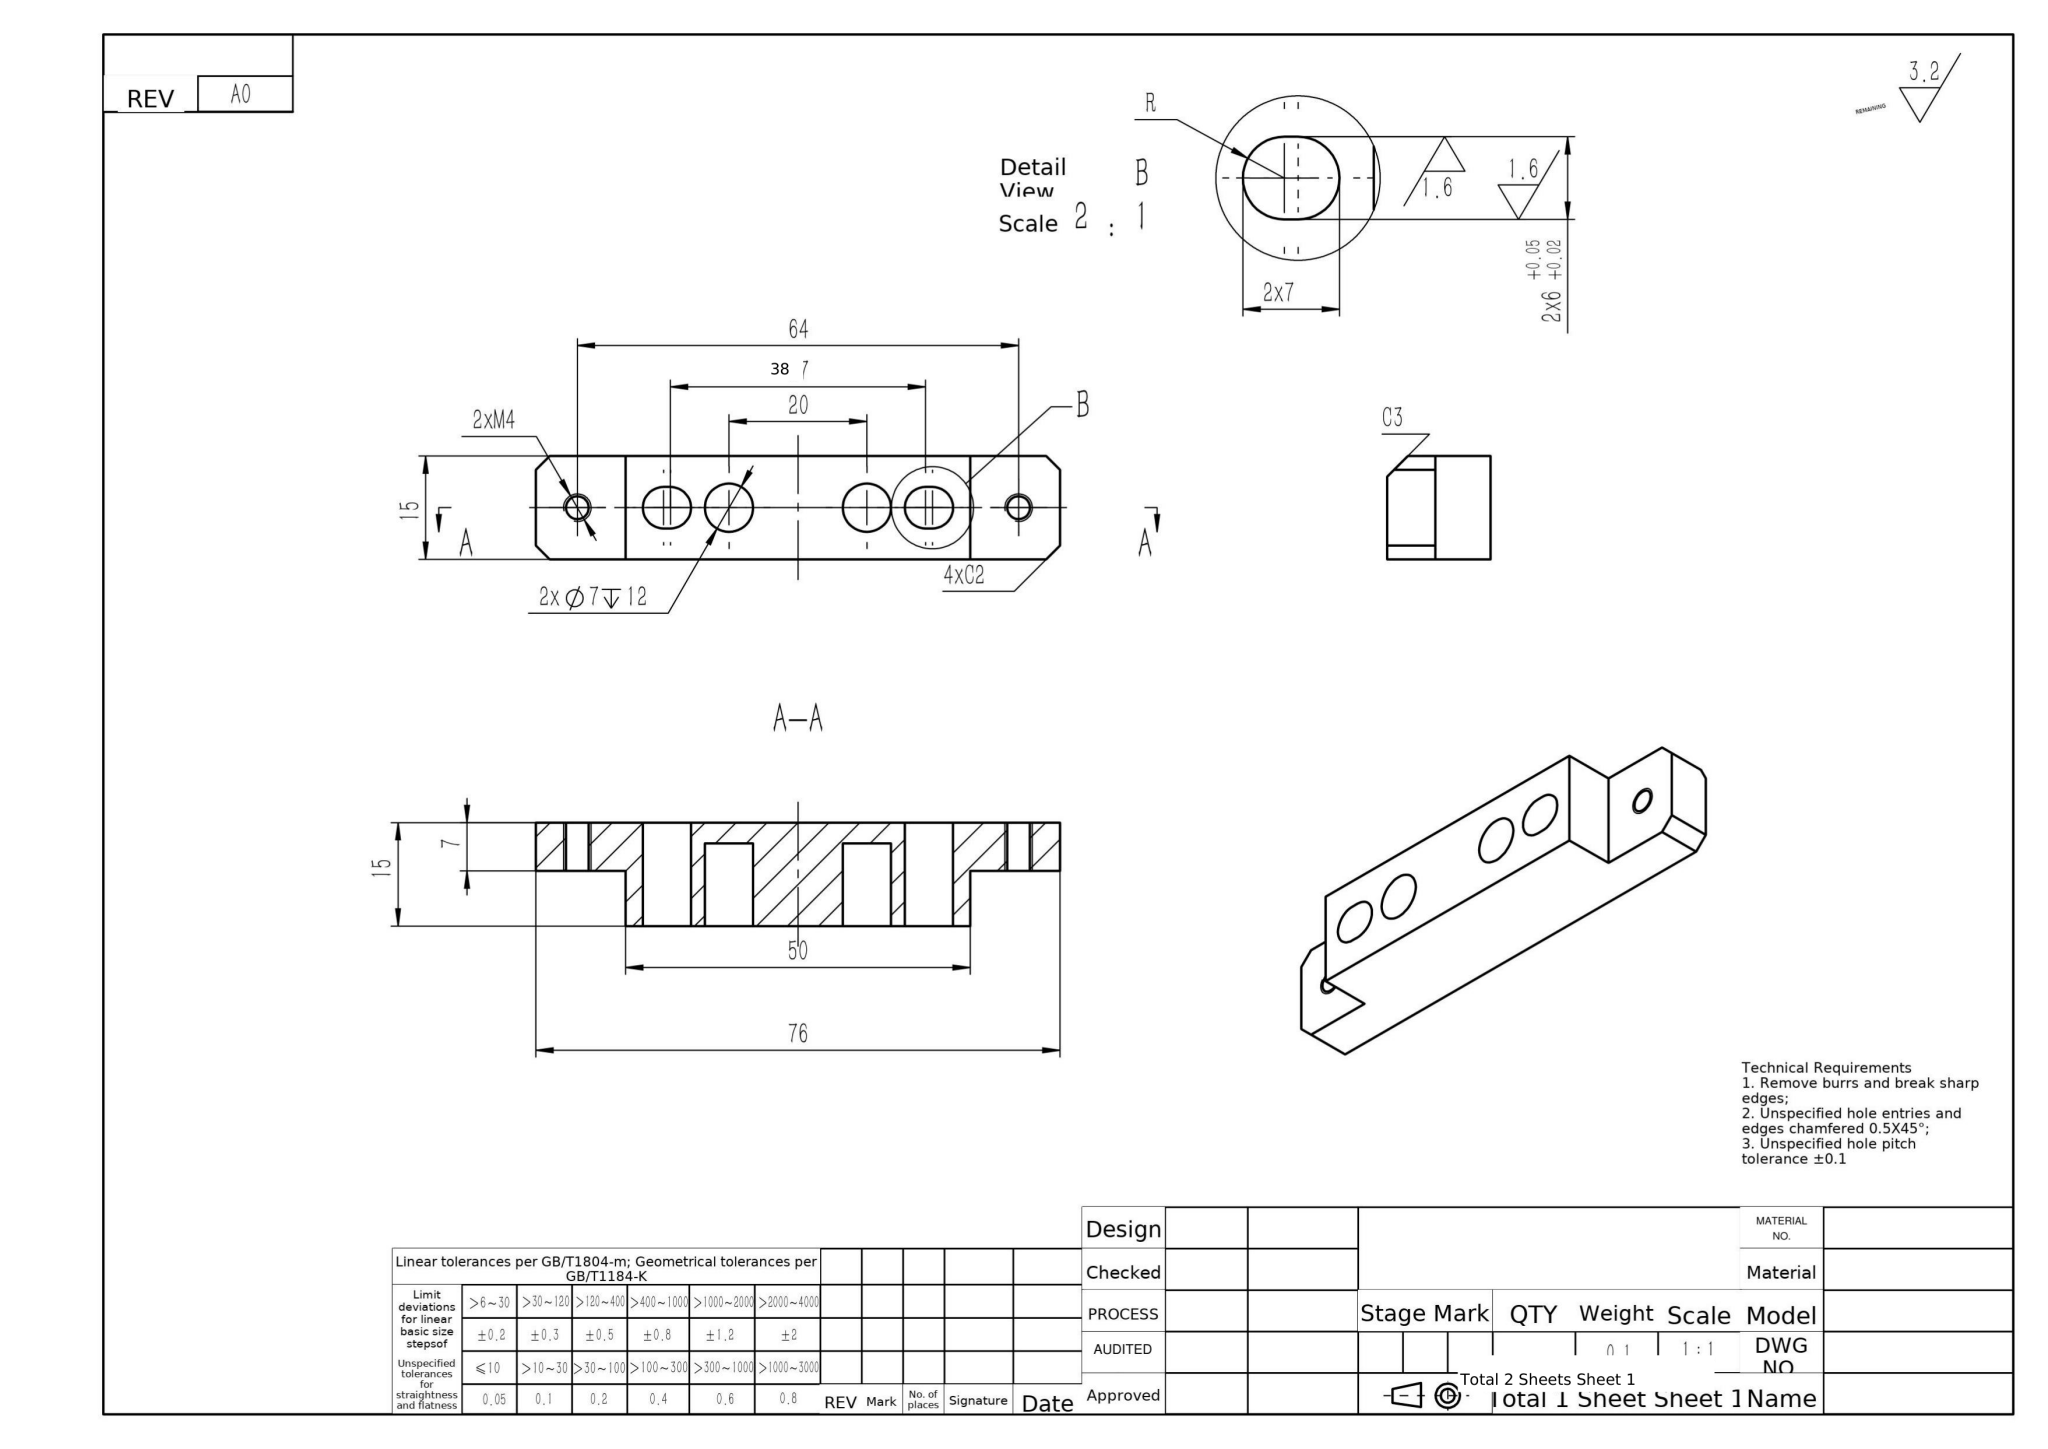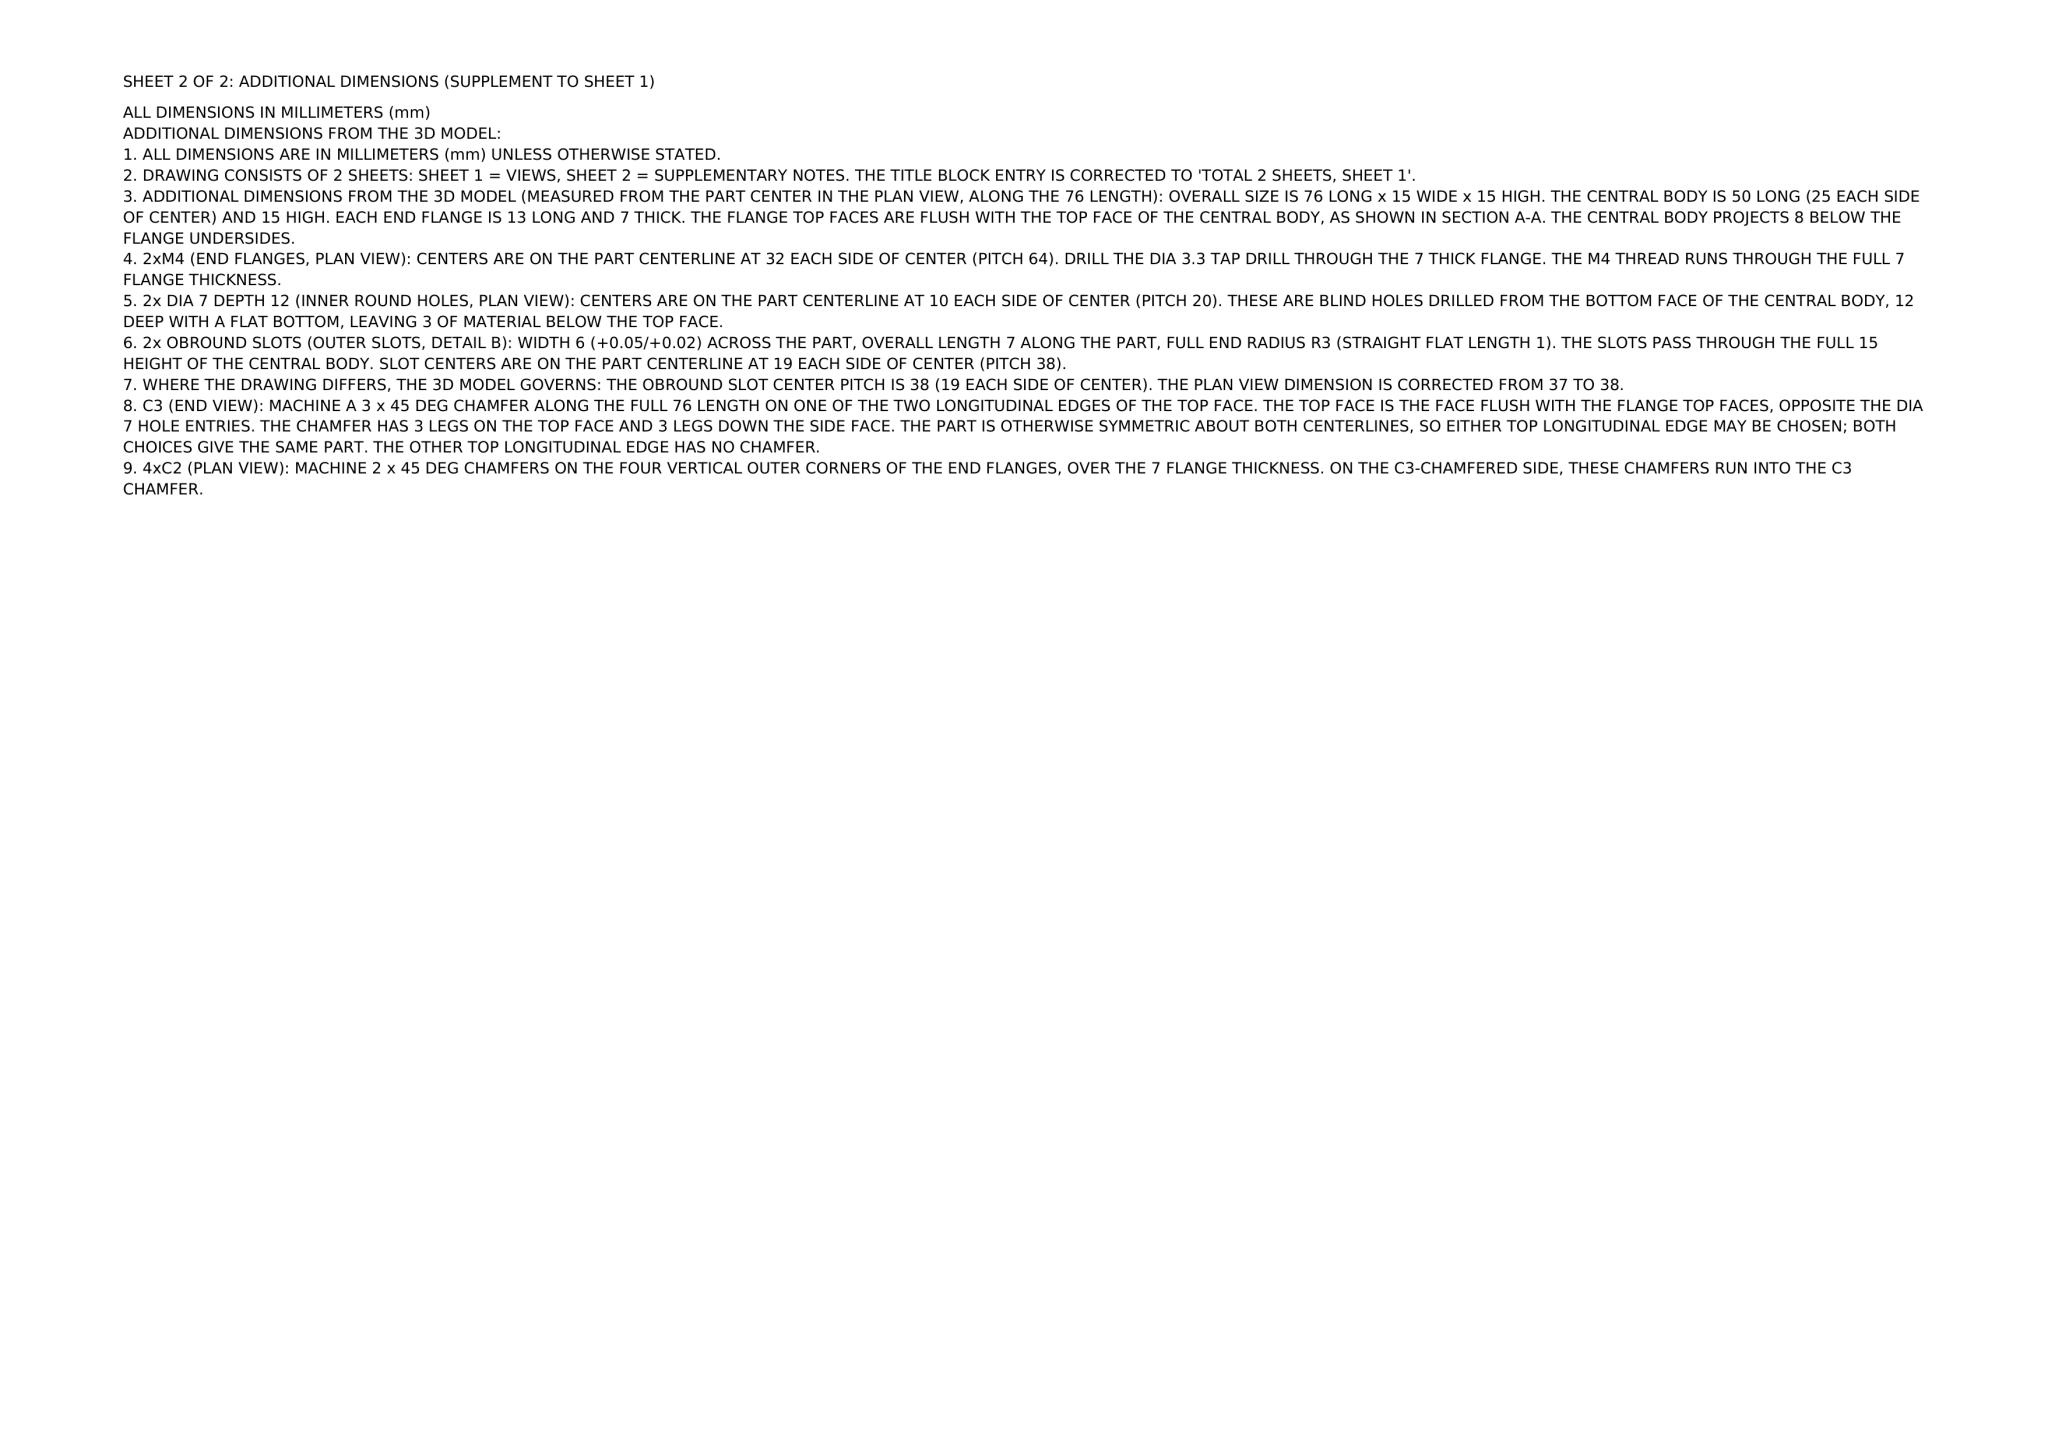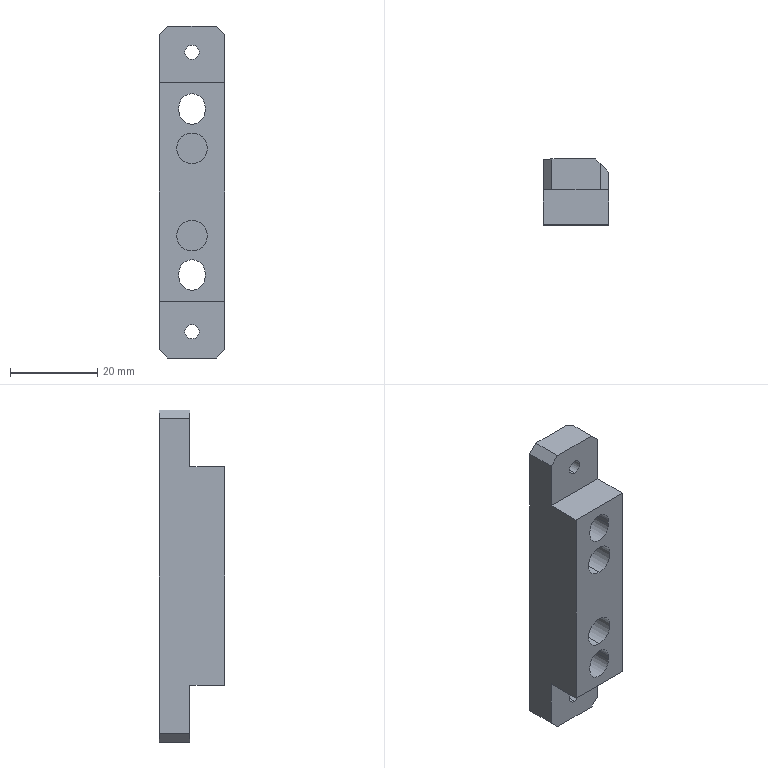Part | NX | mm | Stepped Four-Oval Bore Bracket | 1 solid | 35 faces | box 15 x 15 x 76 mm | volume 11520 mm3 | plane 21 | cylinder 14 | commonest cylinder face diameters 6 x6 3.3 x4 7 x4